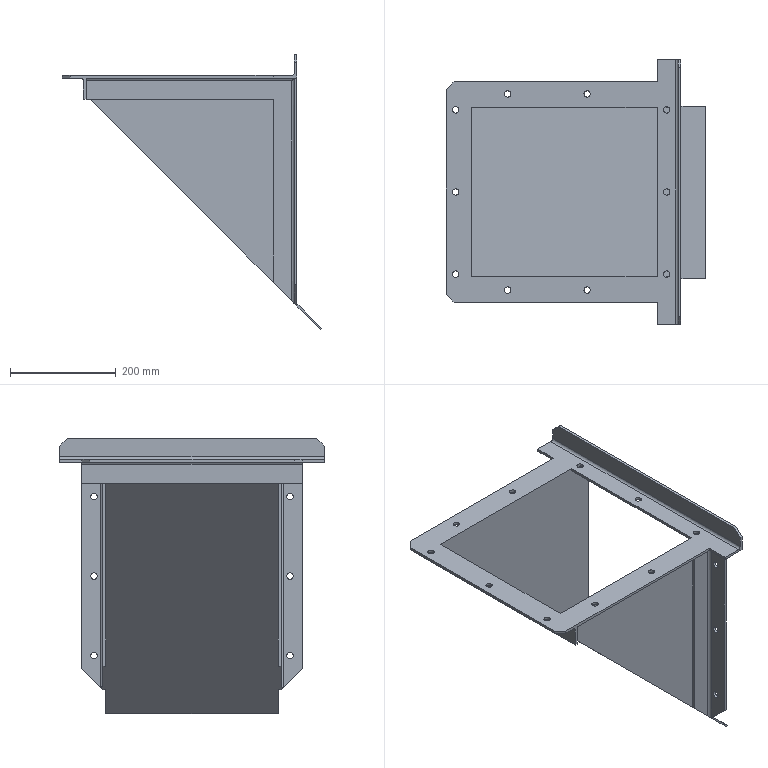Component | SolidWorks | Inlet-1 | 1 solid | 87 faces | box 489.99 x 500 x 519.87 mm | volume 2237972 mm3 | plane 49 | cylinder 38 | commonest cylinder face diameters 12 x32 10 x6
build123d program:
from build123d import *

# Parameters (mm, degrees)
BOSS_EXTRUDE1_DEPTH = 163
SHELL1_T            = -3
BOSS_EXTRUDE2_DEPTH = 208
BOSS_EXTRUDE3_DEPTH = 398
BOSS_EXTRUDE4_START = -3
BOSS_EXTRUDE4_DEPTH = 326
BOSS_EXTRUDE5_DEPTH = 250
BOSS_EXTRUDE6_REACH = 592.351
CHAMFER1_SIZE       = 15
CUT_EXTRUDE1_DEPTH  = 500
SKETCH8_R           = 6
CUT_EXTRUDE2_DEPTH  = 500
CHAMFER2_SIZE       = 15
SKETCH9_R           = 6
CUT_EXTRUDE3_DEPTH  = 10


with BuildPart() as part:
    # Sketch1 → Boss-Extrude1 (new, symmetric)
    with BuildSketch(Plane.XY):
        Polygon((-199, 0), (-199, -37), (199, -435), (199, 0), align=None)
    extrude(amount=BOSS_EXTRUDE1_DEPTH, both=True)

    # Shell1
    shell1_openings = [part.faces().sort_by_distance(p)[0] for p in [
        (199, -217.5, 0),
        (0, 0, 0),
    ]]
    offset(amount=SHELL1_T, openings=shell1_openings, kind=Kind.INTERSECTION)

    # Sketch2 → Boss-Extrude2 (add, symmetric)
    with BuildSketch(Plane.XY):
        with BuildLine():
            Line((-199, 0), (-244, 0))
            Line((-244, 0), (-244, -5))
            Line((-244, -5), (-209, -5))
            ThreePointArc((-209, -5), (-205.464, -6.464), (-204, -10))
            Line((-204, -10), (-204, -45))
            Line((-204, -45), (-199, -45))
            Line((-199, -45), (-199, 0))
        make_face()
    extrude(amount=BOSS_EXTRUDE2_DEPTH, both=True)

    # Sketch3 → Boss-Extrude3 (add)
    with BuildSketch(Plane(origin=(-199, 0, 0), x_dir=(0, 0, -1), z_dir=(1, 0, 0))):
        with BuildLine():
            Line((-208, 0), (-163, 0))
            Line((-163, 0), (-163, -45))
            Line((-163, -45), (-168, -45))
            Line((-168, -45), (-168, -10))
            ThreePointArc((-168, -10), (-169.464, -6.464), (-173, -5))
            Line((-173, -5), (-208, -5))
            Line((-208, -5), (-208, 0))
        make_face()
        with BuildLine():
            Line((208, -5), (208, 0))
            Line((208, 0), (163, 0))
            Line((163, 0), (163, -45))
            Line((163, -45), (168, -45))
            Line((168, -45), (168, -10))
            ThreePointArc((168, -10), (169.464, -6.464), (173, -5))
            Line((173, -5), (208, -5))
        make_face()
    extrude(amount=BOSS_EXTRUDE3_DEPTH)

    # Sketch4 → Boss-Extrude4 (add)
    with BuildSketch(Plane.XY.offset(-160).offset(BOSS_EXTRUDE4_START)):
        Polygon((188.334, -424.334), (243.871, -479.871), (245.992, -477.749), (190.456, -422.213), align=None)
    extrude(amount=BOSS_EXTRUDE4_DEPTH)

    # Sketch5 → Boss-Extrude5 (add, symmetric)
    with BuildSketch(Plane.XY):
        with BuildLine():
            Line((154, 0), (154, -5))
            Line((154, -5), (199, -5))
            Line((199, -5), (199, 40))
            Line((199, 40), (194, 40))
            Line((194, 40), (194, 5))
            ThreePointArc((194, 5), (192.536, 1.464), (189, 0))
            Line((189, 0), (154, 0))
        make_face()
    extrude(amount=BOSS_EXTRUDE5_DEPTH, both=True)

    # Boss-Extrude6: up to this plane
    boss_extrude6_end = Plane(origin=(-199, -37, 163), z_dir=(0.7071, 0.7071, 0))
    # Sketch6 → Boss-Extrude6 (add, up to the surface)
    with BuildSketch(Plane.XZ.offset(5), mode=Mode.PRIVATE) as boss_extrude6_sk1:
        with BuildLine():
            Line((154, 163), (199, 163))
            Line((199, 163), (199, 208))
            Line((199, 208), (194, 208))
            Line((194, 208), (194, 173))
            ThreePointArc((194, 173), (192.536, 169.464), (189, 168))
            Line((189, 168), (154, 168))
            Line((154, 168), (154, 163))
        make_face()
    boss_extrude6_tool1 = split(extrude(boss_extrude6_sk1.sketch, amount=BOSS_EXTRUDE6_REACH, mode=Mode.PRIVATE), bisect_by=boss_extrude6_end, keep=Keep.BOTH, mode=Mode.PRIVATE)
    add(boss_extrude6_tool1.solids().sort_by_distance((176.5, -5, 163.636))[0])
    # Sketch6 → Boss-Extrude6 (add, up to the surface)
    with BuildSketch(Plane.XZ.offset(5), mode=Mode.PRIVATE) as boss_extrude6_sk2:
        with BuildLine():
            Line((154, -168), (154, -163))
            Line((154, -163), (199, -163))
            Line((199, -163), (199, -208))
            Line((199, -208), (194, -208))
            Line((194, -208), (194, -173))
            ThreePointArc((194, -173), (192.536, -169.464), (189, -168))
            Line((189, -168), (154, -168))
        make_face()
    boss_extrude6_tool2 = split(extrude(boss_extrude6_sk2.sketch, amount=BOSS_EXTRUDE6_REACH, mode=Mode.PRIVATE), bisect_by=boss_extrude6_end, keep=Keep.BOTH, mode=Mode.PRIVATE)
    add(boss_extrude6_tool2.solids().sort_by_distance((154.636, -5, -165.5))[0])

    # Chamfer1
    chamfer1_edges = [part.edges().sort_by_distance(p)[0] for p in [
        (196.5, 40, -250),
        (196.5, 40, 250),
    ]]
    chamfer(chamfer1_edges, length=CHAMFER1_SIZE)

    # Sketch7 → Cut-Extrude1 (cut)
    with BuildSketch(Plane.ZY.offset(-194)):
        Polygon((-168, -435), (-208, -395), (-208, -435), align=None)
        Polygon((208, -435), (168, -435), (208, -395), align=None)
    extrude(amount=-CUT_EXTRUDE1_DEPTH, mode=Mode.SUBTRACT)

    # Sketch8 → Cut-Extrude2 (cut)
    with BuildSketch(Plane.ZY.offset(-194)):
        with Locations((-185, -70)):
            Circle(SKETCH8_R)
        with Locations((-185, -370)):
            Circle(SKETCH8_R)
        with Locations((-185, -220)):
            Circle(SKETCH8_R)
        with Locations((185, -370)):
            Circle(SKETCH8_R)
        with Locations((185, -220)):
            Circle(SKETCH8_R)
        with Locations((185, -70)):
            Circle(SKETCH8_R)
    extrude(amount=-CUT_EXTRUDE2_DEPTH, mode=Mode.SUBTRACT)

    # Chamfer2
    chamfer2_edges = [part.edges().sort_by_distance(p)[0] for p in [
        (-244, -2.5, -208),
        (-244, -2.5, 208),
    ]]
    chamfer(chamfer2_edges, length=CHAMFER2_SIZE)

    # Sketch9 → Cut-Extrude3 (cut)
    with BuildSketch(Plane(origin=(0, 0, 0), x_dir=(1, 0, 0), z_dir=(0, 1, 0))):
        with Locations(Location((172, -155, 0), (0, 0, 236.443))):
            Circle(SKETCH9_R)
        with Locations(Location((-226, 0, 0), (0, 0, 180))):
            Circle(SKETCH9_R)
        with Locations(Location((172, 155, 0), (0, 0, 123.557))):
            Circle(SKETCH9_R)
        with Locations(Location((-128, 185, 0), (0, 0, 180))):
            Circle(SKETCH9_R)
        with Locations(Location((22, 185, 0), (0, 0, 180))):
            Circle(SKETCH9_R)
        with Locations(Location((172, 0, 0), (0, 0, 270))):
            Circle(SKETCH9_R)
        with Locations(Location((22, -185, 0), (0, 0, 270))):
            Circle(SKETCH9_R)
        with Locations(Location((-128, -185, 0), (0, 0, 270))):
            Circle(SKETCH9_R)
        with Locations(Location((-226, 155, 0), (0, 0, 180))):
            Circle(SKETCH9_R)
        with Locations(Location((-226, -155, 0), (0, 0, 180))):
            Circle(SKETCH9_R)
    extrude(amount=-CUT_EXTRUDE3_DEPTH, mode=Mode.SUBTRACT)


solid = part.part

# Placed as in the assembly
solid = solid.moved(Location((-762, 0, 240), (90, 0, 0)))